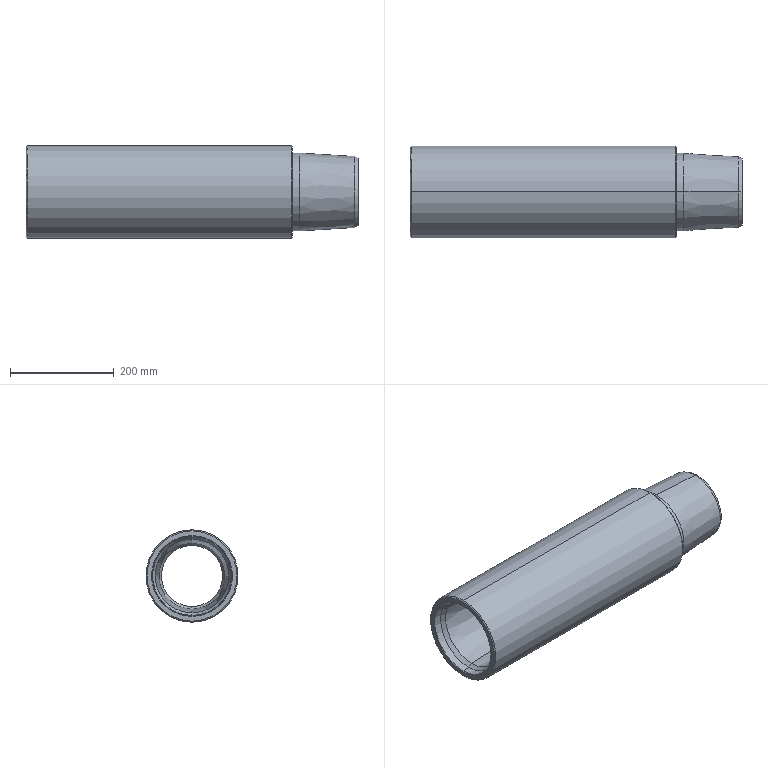Component | SolidWorks | 216OuterTube-1_SpringClipChamber-1 | 1 solid | 34 faces | box 640 x 178 x 178 mm | volume 7081697 mm3 | cone 20 | cylinder 10 | plane 4 | commonest cylinder face diameters 118 x4 150 x2 128 x2 178 x2 | material Alloy Steel
build123d program:
from build123d import *


with BuildPart() as part:
    # Model → Revolve1 (revolve)
    with BuildSketch(Plane.XY, mode=Mode.PRIVATE) as revolve1_sk:
        Polygon((512.079, 89), (3.079, 89), (1.079, 87), (1.079, 77.957), (2.077, 76.896), (17.079, 75.978), (25.583, 71.068), (143.001, 63.886), (151.465, 59), (341.079, 59), (341.079, 64), (421.079, 64), (439.739, 59), (641.079, 59), (641.079, 65.053), (635.079, 68.517), (529.079, 75), (514.079, 75), (514.079, 87), align=None)
    revolve(revolve1_sk.sketch.rotate(Axis((0, 0, 0), (1, 0, 0)), 90), axis=Axis((0, 0, 0), (1, 0, 0)))


solid = part.part
STEP:
#1=COLOUR_RGB('',0.7922,0.8196,0.9333);
#2=FILL_AREA_STYLE_COLOUR('',#1);
#3=FILL_AREA_STYLE('',(#2));
#4=SURFACE_STYLE_FILL_AREA(#3);
#5=SURFACE_SIDE_STYLE('',(#4));
#6=SURFACE_STYLE_USAGE(.BOTH.,#5);
#7=PRESENTATION_STYLE_ASSIGNMENT((#6));
#8=CARTESIAN_POINT('',(20.83,-0.,2.953));
#9=VERTEX_POINT('',#8);
#10=CARTESIAN_POINT('',(20.83,0.,-2.953));
#11=VERTEX_POINT('',#10);
#12=CARTESIAN_POINT('',(20.83,-0.,0.));
#13=DIRECTION('',(-1.,0.,0.));
#14=DIRECTION('',(0.,0.,1.));
#15=AXIS2_PLACEMENT_3D('',#12,#13,#14);
#16=CIRCLE('',#15,2.953);
#17=EDGE_CURVE('',#9,#11,#16,.T.);
#18=ORIENTED_EDGE('',*,*,#17,.T.);
#19=CARTESIAN_POINT('',(20.239,0.,-2.953));
#20=VERTEX_POINT('',#19);
#21=CARTESIAN_POINT('',(-0.,0.,-2.953));
#22=DIRECTION('',(-1.,0.,0.));
#23=VECTOR('',#22,39.37);
#24=LINE('',#21,#23);
#25=EDGE_CURVE('',#11,#20,#24,.T.);
#26=ORIENTED_EDGE('',*,*,#25,.T.);
#27=CARTESIAN_POINT('',(20.239,-0.,2.953));
#28=VERTEX_POINT('',#27);
#29=CARTESIAN_POINT('',(20.239,-0.,0.));
#30=DIRECTION('',(-1.,0.,0.));
#31=DIRECTION('',(0.,0.,1.));
#32=AXIS2_PLACEMENT_3D('',#29,#30,#31);
#33=CIRCLE('',#32,2.953);
#34=EDGE_CURVE('',#28,#20,#33,.T.);
#35=ORIENTED_EDGE('',*,*,#34,.F.);
#36=CARTESIAN_POINT('',(-0.,-0.,2.953));
#37=DIRECTION('',(-1.,0.,0.));
#38=VECTOR('',#37,39.37);
#39=LINE('',#36,#38);
#40=EDGE_CURVE('',#9,#28,#39,.T.);
#41=ORIENTED_EDGE('',*,*,#40,.F.);
#42=EDGE_LOOP('',(#18,#26,#35,#41));
#43=FACE_OUTER_BOUND('',#42,.T.);
#44=CARTESIAN_POINT('',(-0.,-0.,0.));
#45=DIRECTION('',(-1.,0.,0.));
#46=DIRECTION('',(0.,0.,1.));
#47=AXIS2_PLACEMENT_3D('',#44,#45,#46);
#48=CYLINDRICAL_SURFACE('',#47,2.953);
#49=ADVANCED_FACE('',(#43),#48,.T.);
#50=CARTESIAN_POINT('',(25.003,-0.,2.698));
#51=VERTEX_POINT('',#50);
#52=CARTESIAN_POINT('',(25.003,0.,-2.698));
#53=VERTEX_POINT('',#52);
#54=CARTESIAN_POINT('',(25.003,-0.,0.));
#55=DIRECTION('',(-1.,0.,0.));
#56=DIRECTION('',(0.,0.,1.));
#57=AXIS2_PLACEMENT_3D('',#54,#55,#56);
#58=CIRCLE('',#57,2.698);
#59=EDGE_CURVE('',#51,#53,#58,.T.);
#60=ORIENTED_EDGE('',*,*,#59,.T.);
#61=CARTESIAN_POINT('',(25.003,0.,-2.698));
#62=DIRECTION('',(-0.9981,0.,-0.06105));
#63=VECTOR('',#62,39.37);
#64=LINE('',#61,#63);
#65=EDGE_CURVE('',#53,#11,#64,.T.);
#66=ORIENTED_EDGE('',*,*,#65,.T.);
#67=ORIENTED_EDGE('',*,*,#17,.F.);
#68=CARTESIAN_POINT('',(25.003,-0.,2.698));
#69=DIRECTION('',(-0.9981,0.,0.06105));
#70=VECTOR('',#69,39.37);
#71=LINE('',#68,#70);
#72=EDGE_CURVE('',#51,#9,#71,.T.);
#73=ORIENTED_EDGE('',*,*,#72,.F.);
#74=EDGE_LOOP('',(#60,#66,#67,#73));
#75=FACE_OUTER_BOUND('',#74,.T.);
#76=CARTESIAN_POINT('',(25.003,-0.,0.));
#77=DIRECTION('',(-1.,0.,0.));
#78=DIRECTION('',(0.,0.,1.));
#79=AXIS2_PLACEMENT_3D('',#76,#77,#78);
#80=CONICAL_SURFACE('',#79,2.698,0.06109);
#81=ADVANCED_FACE('',(#75),#80,.T.);
#82=CARTESIAN_POINT('',(25.239,-0.,2.561));
#83=VERTEX_POINT('',#82);
#84=CARTESIAN_POINT('',(25.239,0.,-2.561));
#85=VERTEX_POINT('',#84);
#86=CARTESIAN_POINT('',(25.239,-0.,0.));
#87=DIRECTION('',(-1.,0.,0.));
#88=DIRECTION('',(0.,0.,1.));
#89=AXIS2_PLACEMENT_3D('',#86,#87,#88);
#90=CIRCLE('',#89,2.561);
#91=EDGE_CURVE('',#83,#85,#90,.T.);
#92=ORIENTED_EDGE('',*,*,#91,.T.);
#93=CARTESIAN_POINT('',(25.003,0.,-2.698));
#94=DIRECTION('',(-0.866,0.,-0.5));
#95=VECTOR('',#94,39.37);
#96=LINE('',#93,#95);
#97=EDGE_CURVE('',#85,#53,#96,.T.);
#98=ORIENTED_EDGE('',*,*,#97,.T.);
#99=ORIENTED_EDGE('',*,*,#59,.F.);
#100=CARTESIAN_POINT('',(25.003,-0.,2.698));
#101=DIRECTION('',(-0.866,0.,0.5));
#102=VECTOR('',#101,39.37);
#103=LINE('',#100,#102);
#104=EDGE_CURVE('',#83,#51,#103,.T.);
#105=ORIENTED_EDGE('',*,*,#104,.F.);
#106=EDGE_LOOP('',(#92,#98,#99,#105));
#107=FACE_OUTER_BOUND('',#106,.T.);
#108=CARTESIAN_POINT('',(25.003,-0.,0.));
#109=DIRECTION('',(-1.,0.,0.));
#110=DIRECTION('',(0.,0.,1.));
#111=AXIS2_PLACEMENT_3D('',#108,#109,#110);
#112=CONICAL_SURFACE('',#111,2.698,0.5236);
#113=ADVANCED_FACE('',(#107),#112,.T.);
#114=CARTESIAN_POINT('',(25.239,0.,-2.323));
#115=VERTEX_POINT('',#114);
#116=CARTESIAN_POINT('',(25.239,-0.,2.323));
#117=VERTEX_POINT('',#116);
#118=CARTESIAN_POINT('',(25.239,-0.,0.));
#119=DIRECTION('',(-1.,0.,0.));
#120=DIRECTION('',(0.,0.,1.));
#121=AXIS2_PLACEMENT_3D('',#118,#119,#120);
#122=CIRCLE('',#121,2.323);
#123=EDGE_CURVE('',#115,#117,#122,.T.);
#124=ORIENTED_EDGE('',*,*,#123,.F.);
#125=CARTESIAN_POINT('',(17.313,0.,-2.323));
#126=VERTEX_POINT('',#125);
#127=CARTESIAN_POINT('',(-0.,0.,-2.323));
#128=DIRECTION('',(-1.,0.,0.));
#129=VECTOR('',#128,39.37);
#130=LINE('',#127,#129);
#131=EDGE_CURVE('',#115,#126,#130,.T.);
#132=ORIENTED_EDGE('',*,*,#131,.T.);
#133=CARTESIAN_POINT('',(17.313,-0.,2.323));
#134=VERTEX_POINT('',#133);
#135=CARTESIAN_POINT('',(17.313,-0.,0.));
#136=DIRECTION('',(-1.,0.,0.));
#137=DIRECTION('',(0.,0.,1.));
#138=AXIS2_PLACEMENT_3D('',#135,#136,#137);
#139=CIRCLE('',#138,2.323);
#140=EDGE_CURVE('',#126,#134,#139,.T.);
#141=ORIENTED_EDGE('',*,*,#140,.T.);
#142=CARTESIAN_POINT('',(-0.,-0.,2.323));
#143=DIRECTION('',(-1.,0.,0.));
#144=VECTOR('',#143,39.37);
#145=LINE('',#142,#144);
#146=EDGE_CURVE('',#117,#134,#145,.T.);
#147=ORIENTED_EDGE('',*,*,#146,.F.);
#148=EDGE_LOOP('',(#124,#132,#141,#147));
#149=FACE_OUTER_BOUND('',#148,.T.);
#150=CARTESIAN_POINT('',(-0.,-0.,0.));
#151=DIRECTION('',(-1.,0.,0.));
#152=DIRECTION('',(0.,0.,1.));
#153=AXIS2_PLACEMENT_3D('',#150,#151,#152);
#154=CYLINDRICAL_SURFACE('',#153,2.323);
#155=ADVANCED_FACE('',(#149),#154,.F.);
#156=ORIENTED_EDGE('',*,*,#140,.F.);
#157=CARTESIAN_POINT('',(16.578,0.,-2.52));
#158=VERTEX_POINT('',#157);
#159=CARTESIAN_POINT('',(16.578,0.,-2.52));
#160=DIRECTION('',(-0.9659,0.,-0.2588));
#161=VECTOR('',#160,39.37);
#162=LINE('',#159,#161);
#163=EDGE_CURVE('',#126,#158,#162,.T.);
#164=ORIENTED_EDGE('',*,*,#163,.T.);
#165=CARTESIAN_POINT('',(16.578,-0.,2.52));
#166=VERTEX_POINT('',#165);
#167=CARTESIAN_POINT('',(16.578,-0.,0.));
#168=DIRECTION('',(-1.,0.,0.));
#169=DIRECTION('',(0.,0.,1.));
#170=AXIS2_PLACEMENT_3D('',#167,#168,#169);
#171=CIRCLE('',#170,2.52);
#172=EDGE_CURVE('',#158,#166,#171,.T.);
#173=ORIENTED_EDGE('',*,*,#172,.T.);
#174=CARTESIAN_POINT('',(16.578,-0.,2.52));
#175=DIRECTION('',(-0.9659,0.,0.2588));
#176=VECTOR('',#175,39.37);
#177=LINE('',#174,#176);
#178=EDGE_CURVE('',#134,#166,#177,.T.);
#179=ORIENTED_EDGE('',*,*,#178,.F.);
#180=EDGE_LOOP('',(#156,#164,#173,#179));
#181=FACE_OUTER_BOUND('',#180,.T.);
#182=CARTESIAN_POINT('',(16.578,-0.,0.));
#183=DIRECTION('',(-1.,0.,0.));
#184=DIRECTION('',(0.,0.,1.));
#185=AXIS2_PLACEMENT_3D('',#182,#183,#184);
#186=CONICAL_SURFACE('',#185,2.52,0.2618);
#187=ADVANCED_FACE('',(#181),#186,.F.);
#188=ORIENTED_EDGE('',*,*,#172,.F.);
#189=CARTESIAN_POINT('',(13.428,0.,-2.52));
#190=VERTEX_POINT('',#189);
#191=CARTESIAN_POINT('',(-0.,0.,-2.52));
#192=DIRECTION('',(-1.,0.,0.));
#193=VECTOR('',#192,39.37);
#194=LINE('',#191,#193);
#195=EDGE_CURVE('',#158,#190,#194,.T.);
#196=ORIENTED_EDGE('',*,*,#195,.T.);
#197=CARTESIAN_POINT('',(13.428,-0.,2.52));
#198=VERTEX_POINT('',#197);
#199=CARTESIAN_POINT('',(13.428,-0.,0.));
#200=DIRECTION('',(-1.,0.,0.));
#201=DIRECTION('',(0.,0.,1.));
#202=AXIS2_PLACEMENT_3D('',#199,#200,#201);
#203=CIRCLE('',#202,2.52);
#204=EDGE_CURVE('',#190,#198,#203,.T.);
#205=ORIENTED_EDGE('',*,*,#204,.T.);
#206=CARTESIAN_POINT('',(-0.,-0.,2.52));
#207=DIRECTION('',(-1.,0.,0.));
#208=VECTOR('',#207,39.37);
#209=LINE('',#206,#208);
#210=EDGE_CURVE('',#166,#198,#209,.T.);
#211=ORIENTED_EDGE('',*,*,#210,.F.);
#212=EDGE_LOOP('',(#188,#196,#205,#211));
#213=FACE_OUTER_BOUND('',#212,.T.);
#214=CARTESIAN_POINT('',(-0.,-0.,0.));
#215=DIRECTION('',(-1.,0.,0.));
#216=DIRECTION('',(0.,0.,1.));
#217=AXIS2_PLACEMENT_3D('',#214,#215,#216);
#218=CYLINDRICAL_SURFACE('',#217,2.52);
#219=ADVANCED_FACE('',(#213),#218,.F.);
#220=CARTESIAN_POINT('',(13.428,0.,-2.323));
#221=VERTEX_POINT('',#220);
#222=CARTESIAN_POINT('',(13.428,-0.,2.323));
#223=VERTEX_POINT('',#222);
#224=CARTESIAN_POINT('',(13.428,-0.,0.));
#225=DIRECTION('',(-1.,0.,0.));
#226=DIRECTION('',(0.,0.,1.));
#227=AXIS2_PLACEMENT_3D('',#224,#225,#226);
#228=CIRCLE('',#227,2.323);
#229=EDGE_CURVE('',#221,#223,#228,.T.);
#230=ORIENTED_EDGE('',*,*,#229,.F.);
#231=CARTESIAN_POINT('',(5.963,0.,-2.323));
#232=VERTEX_POINT('',#231);
#233=CARTESIAN_POINT('',(-0.,0.,-2.323));
#234=DIRECTION('',(-1.,0.,0.));
#235=VECTOR('',#234,39.37);
#236=LINE('',#233,#235);
#237=EDGE_CURVE('',#221,#232,#236,.T.);
#238=ORIENTED_EDGE('',*,*,#237,.T.);
#239=CARTESIAN_POINT('',(5.963,-0.,2.323));
#240=VERTEX_POINT('',#239);
#241=CARTESIAN_POINT('',(5.963,-0.,0.));
#242=DIRECTION('',(-1.,0.,0.));
#243=DIRECTION('',(0.,0.,1.));
#244=AXIS2_PLACEMENT_3D('',#241,#242,#243);
#245=CIRCLE('',#244,2.323);
#246=EDGE_CURVE('',#232,#240,#245,.T.);
#247=ORIENTED_EDGE('',*,*,#246,.T.);
#248=CARTESIAN_POINT('',(-0.,-0.,2.323));
#249=DIRECTION('',(-1.,0.,0.));
#250=VECTOR('',#249,39.37);
#251=LINE('',#248,#250);
#252=EDGE_CURVE('',#223,#240,#251,.T.);
#253=ORIENTED_EDGE('',*,*,#252,.F.);
#254=EDGE_LOOP('',(#230,#238,#247,#253));
#255=FACE_OUTER_BOUND('',#254,.T.);
#256=CARTESIAN_POINT('',(-0.,-0.,0.));
#257=DIRECTION('',(-1.,0.,0.));
#258=DIRECTION('',(0.,0.,1.));
#259=AXIS2_PLACEMENT_3D('',#256,#257,#258);
#260=CYLINDRICAL_SURFACE('',#259,2.323);
#261=ADVANCED_FACE('',(#255),#260,.F.);
#262=ORIENTED_EDGE('',*,*,#246,.F.);
#263=CARTESIAN_POINT('',(5.63,0.,-2.515));
#264=VERTEX_POINT('',#263);
#265=CARTESIAN_POINT('',(5.63,0.,-2.515));
#266=DIRECTION('',(-0.866,0.,-0.5));
#267=VECTOR('',#266,39.37);
#268=LINE('',#265,#267);
#269=EDGE_CURVE('',#232,#264,#268,.T.);
#270=ORIENTED_EDGE('',*,*,#269,.T.);
#271=CARTESIAN_POINT('',(5.63,-0.,2.515));
#272=VERTEX_POINT('',#271);
#273=CARTESIAN_POINT('',(5.63,-0.,0.));
#274=DIRECTION('',(-1.,0.,0.));
#275=DIRECTION('',(0.,0.,1.));
#276=AXIS2_PLACEMENT_3D('',#273,#274,#275);
#277=CIRCLE('',#276,2.515);
#278=EDGE_CURVE('',#264,#272,#277,.T.);
#279=ORIENTED_EDGE('',*,*,#278,.T.);
#280=CARTESIAN_POINT('',(5.63,-0.,2.515));
#281=DIRECTION('',(-0.866,0.,0.5));
#282=VECTOR('',#281,39.37);
#283=LINE('',#280,#282);
#284=EDGE_CURVE('',#240,#272,#283,.T.);
#285=ORIENTED_EDGE('',*,*,#284,.F.);
#286=EDGE_LOOP('',(#262,#270,#279,#285));
#287=FACE_OUTER_BOUND('',#286,.T.);
#288=CARTESIAN_POINT('',(5.63,-0.,0.));
#289=DIRECTION('',(-1.,0.,0.));
#290=DIRECTION('',(0.,0.,1.));
#291=AXIS2_PLACEMENT_3D('',#288,#289,#290);
#292=CONICAL_SURFACE('',#291,2.515,0.5236);
#293=ADVANCED_FACE('',(#287),#292,.F.);
#294=ORIENTED_EDGE('',*,*,#278,.F.);
#295=CARTESIAN_POINT('',(1.007,0.,-2.798));
#296=VERTEX_POINT('',#295);
#297=CARTESIAN_POINT('',(1.007,0.,-2.798));
#298=DIRECTION('',(-0.9981,0.,-0.06105));
#299=VECTOR('',#298,39.37);
#300=LINE('',#297,#299);
#301=EDGE_CURVE('',#264,#296,#300,.T.);
#302=ORIENTED_EDGE('',*,*,#301,.T.);
#303=CARTESIAN_POINT('',(1.007,-0.,2.798));
#304=VERTEX_POINT('',#303);
#305=CARTESIAN_POINT('',(1.007,-0.,0.));
#306=DIRECTION('',(-1.,0.,0.));
#307=DIRECTION('',(0.,0.,1.));
#308=AXIS2_PLACEMENT_3D('',#305,#306,#307);
#309=CIRCLE('',#308,2.798);
#310=EDGE_CURVE('',#296,#304,#309,.T.);
#311=ORIENTED_EDGE('',*,*,#310,.T.);
#312=CARTESIAN_POINT('',(1.007,-0.,2.798));
#313=DIRECTION('',(-0.9981,0.,0.06105));
#314=VECTOR('',#313,39.37);
#315=LINE('',#312,#314);
#316=EDGE_CURVE('',#272,#304,#315,.T.);
#317=ORIENTED_EDGE('',*,*,#316,.F.);
#318=EDGE_LOOP('',(#294,#302,#311,#317));
#319=FACE_OUTER_BOUND('',#318,.T.);
#320=CARTESIAN_POINT('',(1.007,-0.,0.));
#321=DIRECTION('',(-1.,0.,0.));
#322=DIRECTION('',(0.,0.,1.));
#323=AXIS2_PLACEMENT_3D('',#320,#321,#322);
#324=CONICAL_SURFACE('',#323,2.798,0.06109);
#325=ADVANCED_FACE('',(#319),#324,.F.);
#326=ORIENTED_EDGE('',*,*,#310,.F.);
#327=CARTESIAN_POINT('',(0.6724,0.,-2.991));
#328=VERTEX_POINT('',#327);
#329=CARTESIAN_POINT('',(0.6724,0.,-2.991));
#330=DIRECTION('',(-0.866,0.,-0.5));
#331=VECTOR('',#330,39.37);
#332=LINE('',#329,#331);
#333=EDGE_CURVE('',#296,#328,#332,.T.);
#334=ORIENTED_EDGE('',*,*,#333,.T.);
#335=CARTESIAN_POINT('',(0.6724,-0.,2.991));
#336=VERTEX_POINT('',#335);
#337=CARTESIAN_POINT('',(0.6724,-0.,0.));
#338=DIRECTION('',(-1.,0.,0.));
#339=DIRECTION('',(0.,0.,1.));
#340=AXIS2_PLACEMENT_3D('',#337,#338,#339);
#341=CIRCLE('',#340,2.991);
#342=EDGE_CURVE('',#328,#336,#341,.T.);
#343=ORIENTED_EDGE('',*,*,#342,.T.);
#344=CARTESIAN_POINT('',(0.6724,-0.,2.991));
#345=DIRECTION('',(-0.866,0.,0.5));
#346=VECTOR('',#345,39.37);
#347=LINE('',#344,#346);
#348=EDGE_CURVE('',#304,#336,#347,.T.);
#349=ORIENTED_EDGE('',*,*,#348,.F.);
#350=EDGE_LOOP('',(#326,#334,#343,#349));
#351=FACE_OUTER_BOUND('',#350,.T.);
#352=CARTESIAN_POINT('',(0.6724,-0.,0.));
#353=DIRECTION('',(-1.,0.,0.));
#354=DIRECTION('',(0.,0.,1.));
#355=AXIS2_PLACEMENT_3D('',#352,#353,#354);
#356=CONICAL_SURFACE('',#355,2.991,0.5236);
#357=ADVANCED_FACE('',(#351),#356,.F.);
#358=ORIENTED_EDGE('',*,*,#342,.F.);
#359=CARTESIAN_POINT('',(0.08177,0.,-3.027));
#360=VERTEX_POINT('',#359);
#361=CARTESIAN_POINT('',(0.08177,0.,-3.027));
#362=DIRECTION('',(-0.9981,0.,-0.06105));
#363=VECTOR('',#362,39.37);
#364=LINE('',#361,#363);
#365=EDGE_CURVE('',#328,#360,#364,.T.);
#366=ORIENTED_EDGE('',*,*,#365,.T.);
#367=CARTESIAN_POINT('',(0.08177,-0.,3.027));
#368=VERTEX_POINT('',#367);
#369=CARTESIAN_POINT('',(0.08177,-0.,0.));
#370=DIRECTION('',(-1.,0.,0.));
#371=DIRECTION('',(0.,0.,1.));
#372=AXIS2_PLACEMENT_3D('',#369,#370,#371);
#373=CIRCLE('',#372,3.027);
#374=EDGE_CURVE('',#360,#368,#373,.T.);
#375=ORIENTED_EDGE('',*,*,#374,.T.);
#376=CARTESIAN_POINT('',(0.08177,-0.,3.027));
#377=DIRECTION('',(-0.9981,0.,0.06105));
#378=VECTOR('',#377,39.37);
#379=LINE('',#376,#378);
#380=EDGE_CURVE('',#336,#368,#379,.T.);
#381=ORIENTED_EDGE('',*,*,#380,.F.);
#382=EDGE_LOOP('',(#358,#366,#375,#381));
#383=FACE_OUTER_BOUND('',#382,.T.);
#384=CARTESIAN_POINT('',(0.08177,-0.,0.));
#385=DIRECTION('',(-1.,0.,0.));
#386=DIRECTION('',(0.,0.,1.));
#387=AXIS2_PLACEMENT_3D('',#384,#385,#386);
#388=CONICAL_SURFACE('',#387,3.027,0.06109);
#389=ADVANCED_FACE('',(#383),#388,.F.);
#390=ORIENTED_EDGE('',*,*,#374,.F.);
#391=CARTESIAN_POINT('',(0.04247,0.,-3.069));
#392=VERTEX_POINT('',#391);
#393=CARTESIAN_POINT('',(0.04247,0.,-3.069));
#394=DIRECTION('',(-0.6852,0.,-0.7284));
#395=VECTOR('',#394,39.37);
#396=LINE('',#393,#395);
#397=EDGE_CURVE('',#360,#392,#396,.T.);
#398=ORIENTED_EDGE('',*,*,#397,.T.);
#399=CARTESIAN_POINT('',(0.04247,-0.,3.069));
#400=VERTEX_POINT('',#399);
#401=CARTESIAN_POINT('',(0.04247,-0.,0.));
#402=DIRECTION('',(-1.,0.,0.));
#403=DIRECTION('',(0.,0.,1.));
#404=AXIS2_PLACEMENT_3D('',#401,#402,#403);
#405=CIRCLE('',#404,3.069);
#406=EDGE_CURVE('',#392,#400,#405,.T.);
#407=ORIENTED_EDGE('',*,*,#406,.T.);
#408=CARTESIAN_POINT('',(0.04247,-0.,3.069));
#409=DIRECTION('',(-0.6852,0.,0.7284));
#410=VECTOR('',#409,39.37);
#411=LINE('',#408,#410);
#412=EDGE_CURVE('',#368,#400,#411,.T.);
#413=ORIENTED_EDGE('',*,*,#412,.F.);
#414=EDGE_LOOP('',(#390,#398,#407,#413));
#415=FACE_OUTER_BOUND('',#414,.T.);
#416=CARTESIAN_POINT('',(0.04247,-0.,0.));
#417=DIRECTION('',(-1.,0.,0.));
#418=DIRECTION('',(0.,0.,1.));
#419=AXIS2_PLACEMENT_3D('',#416,#417,#418);
#420=CONICAL_SURFACE('',#419,3.069,0.8159);
#421=ADVANCED_FACE('',(#415),#420,.F.);
#422=CARTESIAN_POINT('',(0.04247,0.,3.425));
#423=VERTEX_POINT('',#422);
#424=CARTESIAN_POINT('',(0.04247,-0.,-3.425));
#425=VERTEX_POINT('',#424);
#426=CARTESIAN_POINT('',(0.04247,-0.,0.));
#427=DIRECTION('',(-1.,0.,0.));
#428=DIRECTION('',(0.,0.,1.));
#429=AXIS2_PLACEMENT_3D('',#426,#427,#428);
#430=CIRCLE('',#429,3.425);
#431=EDGE_CURVE('',#423,#425,#430,.T.);
#432=ORIENTED_EDGE('',*,*,#431,.F.);
#433=CARTESIAN_POINT('',(0.1212,-0.,3.504));
#434=VERTEX_POINT('',#433);
#435=CARTESIAN_POINT('',(0.04247,0.,3.425));
#436=DIRECTION('',(0.7071,0.,0.7071));
#437=VECTOR('',#436,39.37);
#438=LINE('',#435,#437);
#439=EDGE_CURVE('',#423,#434,#438,.T.);
#440=ORIENTED_EDGE('',*,*,#439,.T.);
#441=CARTESIAN_POINT('',(0.1212,0.,-3.504));
#442=VERTEX_POINT('',#441);
#443=CARTESIAN_POINT('',(0.1212,-0.,0.));
#444=DIRECTION('',(-1.,0.,0.));
#445=DIRECTION('',(0.,0.,1.));
#446=AXIS2_PLACEMENT_3D('',#443,#444,#445);
#447=CIRCLE('',#446,3.504);
#448=EDGE_CURVE('',#434,#442,#447,.T.);
#449=ORIENTED_EDGE('',*,*,#448,.T.);
#450=CARTESIAN_POINT('',(0.04247,-0.,-3.425));
#451=DIRECTION('',(0.7071,0.,-0.7071));
#452=VECTOR('',#451,39.37);
#453=LINE('',#450,#452);
#454=EDGE_CURVE('',#425,#442,#453,.T.);
#455=ORIENTED_EDGE('',*,*,#454,.F.);
#456=EDGE_LOOP('',(#432,#440,#449,#455));
#457=FACE_OUTER_BOUND('',#456,.T.);
#458=CARTESIAN_POINT('',(0.04247,-0.,0.));
#459=DIRECTION('',(1.,0.,0.));
#460=DIRECTION('',(0.,0.,-1.));
#461=AXIS2_PLACEMENT_3D('',#458,#459,#460);
#462=CONICAL_SURFACE('',#461,3.425,0.7854);
#463=ADVANCED_FACE('',(#457),#462,.T.);
#464=CARTESIAN_POINT('',(20.161,-0.,3.504));
#465=VERTEX_POINT('',#464);
#466=CARTESIAN_POINT('',(20.161,0.,-3.504));
#467=VERTEX_POINT('',#466);
#468=CARTESIAN_POINT('',(20.161,-0.,0.));
#469=DIRECTION('',(-1.,0.,0.));
#470=DIRECTION('',(0.,0.,1.));
#471=AXIS2_PLACEMENT_3D('',#468,#469,#470);
#472=CIRCLE('',#471,3.504);
#473=EDGE_CURVE('',#465,#467,#472,.T.);
#474=ORIENTED_EDGE('',*,*,#473,.T.);
#475=CARTESIAN_POINT('',(-0.,0.,-3.504));
#476=DIRECTION('',(-1.,0.,0.));
#477=VECTOR('',#476,39.37);
#478=LINE('',#475,#477);
#479=EDGE_CURVE('',#467,#442,#478,.T.);
#480=ORIENTED_EDGE('',*,*,#479,.T.);
#481=ORIENTED_EDGE('',*,*,#448,.F.);
#482=CARTESIAN_POINT('',(-0.,-0.,3.504));
#483=DIRECTION('',(-1.,0.,0.));
#484=VECTOR('',#483,39.37);
#485=LINE('',#482,#484);
#486=EDGE_CURVE('',#465,#434,#485,.T.);
#487=ORIENTED_EDGE('',*,*,#486,.F.);
#488=EDGE_LOOP('',(#474,#480,#481,#487));
#489=FACE_OUTER_BOUND('',#488,.T.);
#490=CARTESIAN_POINT('',(-0.,-0.,0.));
#491=DIRECTION('',(-1.,0.,0.));
#492=DIRECTION('',(0.,0.,1.));
#493=AXIS2_PLACEMENT_3D('',#490,#491,#492);
#494=CYLINDRICAL_SURFACE('',#493,3.504);
#495=ADVANCED_FACE('',(#489),#494,.T.);
#496=CARTESIAN_POINT('',(20.239,-0.,3.425));
#497=VERTEX_POINT('',#496);
#498=CARTESIAN_POINT('',(20.239,0.,-3.425));
#499=VERTEX_POINT('',#498);
#500=CARTESIAN_POINT('',(20.239,-0.,0.));
#501=DIRECTION('',(-1.,0.,0.));
#502=DIRECTION('',(0.,0.,1.));
#503=AXIS2_PLACEMENT_3D('',#500,#501,#502);
#504=CIRCLE('',#503,3.425);
#505=EDGE_CURVE('',#497,#499,#504,.T.);
#506=ORIENTED_EDGE('',*,*,#505,.T.);
#507=CARTESIAN_POINT('',(20.239,0.,-3.425));
#508=DIRECTION('',(-0.7071,0.,-0.7071));
#509=VECTOR('',#508,39.37);
#510=LINE('',#507,#509);
#511=EDGE_CURVE('',#499,#467,#510,.T.);
#512=ORIENTED_EDGE('',*,*,#511,.T.);
#513=ORIENTED_EDGE('',*,*,#473,.F.);
#514=CARTESIAN_POINT('',(20.239,-0.,3.425));
#515=DIRECTION('',(-0.7071,0.,0.7071));
#516=VECTOR('',#515,39.37);
#517=LINE('',#514,#516);
#518=EDGE_CURVE('',#497,#465,#517,.T.);
#519=ORIENTED_EDGE('',*,*,#518,.F.);
#520=EDGE_LOOP('',(#506,#512,#513,#519));
#521=FACE_OUTER_BOUND('',#520,.T.);
#522=CARTESIAN_POINT('',(20.239,-0.,0.));
#523=DIRECTION('',(-1.,0.,0.));
#524=DIRECTION('',(0.,0.,1.));
#525=AXIS2_PLACEMENT_3D('',#522,#523,#524);
#526=CONICAL_SURFACE('',#525,3.425,0.7854);
#527=ADVANCED_FACE('',(#521),#526,.T.);
#528=ORIENTED_EDGE('',*,*,#34,.T.);
#529=CARTESIAN_POINT('',(20.239,-0.,0.));
#530=DIRECTION('',(-1.,0.,0.));
#531=DIRECTION('',(0.,0.,1.));
#532=AXIS2_PLACEMENT_3D('',#529,#530,#531);
#533=CIRCLE('',#532,2.953);
#534=EDGE_CURVE('',#20,#28,#533,.T.);
#535=ORIENTED_EDGE('',*,*,#534,.T.);
#536=EDGE_LOOP('',(#528,#535));
#537=FACE_BOUND('',#536,.T.);
#538=ORIENTED_EDGE('',*,*,#505,.F.);
#539=CARTESIAN_POINT('',(20.239,-0.,0.));
#540=DIRECTION('',(-1.,0.,0.));
#541=DIRECTION('',(0.,0.,1.));
#542=AXIS2_PLACEMENT_3D('',#539,#540,#541);
#543=CIRCLE('',#542,3.425);
#544=EDGE_CURVE('',#499,#497,#543,.T.);
#545=ORIENTED_EDGE('',*,*,#544,.F.);
#546=EDGE_LOOP('',(#538,#545));
#547=FACE_OUTER_BOUND('',#546,.T.);
#548=CARTESIAN_POINT('',(20.239,0.,0.));
#549=DIRECTION('',(1.,0.,0.));
#550=DIRECTION('',(0.,0.,-1.));
#551=AXIS2_PLACEMENT_3D('',#548,#549,#550);
#552=PLANE('',#551);
#553=ADVANCED_FACE('',(#537,#547),#552,.T.);
#554=ORIENTED_EDGE('',*,*,#511,.F.);
#555=ORIENTED_EDGE('',*,*,#544,.T.);
#556=ORIENTED_EDGE('',*,*,#518,.T.);
#557=CARTESIAN_POINT('',(20.161,-0.,0.));
#558=DIRECTION('',(-1.,0.,0.));
#559=DIRECTION('',(0.,0.,1.));
#560=AXIS2_PLACEMENT_3D('',#557,#558,#559);
#561=CIRCLE('',#560,3.504);
#562=EDGE_CURVE('',#467,#465,#561,.T.);
#563=ORIENTED_EDGE('',*,*,#562,.F.);
#564=EDGE_LOOP('',(#554,#555,#556,#563));
#565=FACE_OUTER_BOUND('',#564,.T.);
#566=CARTESIAN_POINT('',(20.239,-0.,0.));
#567=DIRECTION('',(-1.,0.,0.));
#568=DIRECTION('',(0.,0.,1.));
#569=AXIS2_PLACEMENT_3D('',#566,#567,#568);
#570=CONICAL_SURFACE('',#569,3.425,0.7854);
#571=ADVANCED_FACE('',(#565),#570,.T.);
#572=ORIENTED_EDGE('',*,*,#479,.F.);
#573=ORIENTED_EDGE('',*,*,#562,.T.);
#574=ORIENTED_EDGE('',*,*,#486,.T.);
#575=CARTESIAN_POINT('',(0.1212,-0.,0.));
#576=DIRECTION('',(-1.,0.,0.));
#577=DIRECTION('',(0.,0.,1.));
#578=AXIS2_PLACEMENT_3D('',#575,#576,#577);
#579=CIRCLE('',#578,3.504);
#580=EDGE_CURVE('',#442,#434,#579,.T.);
#581=ORIENTED_EDGE('',*,*,#580,.F.);
#582=EDGE_LOOP('',(#572,#573,#574,#581));
#583=FACE_OUTER_BOUND('',#582,.T.);
#584=CARTESIAN_POINT('',(-0.,-0.,0.));
#585=DIRECTION('',(-1.,0.,0.));
#586=DIRECTION('',(0.,0.,1.));
#587=AXIS2_PLACEMENT_3D('',#584,#585,#586);
#588=CYLINDRICAL_SURFACE('',#587,3.504);
#589=ADVANCED_FACE('',(#583),#588,.T.);
#590=ORIENTED_EDGE('',*,*,#439,.F.);
#591=CARTESIAN_POINT('',(0.04247,-0.,0.));
#592=DIRECTION('',(-1.,0.,0.));
#593=DIRECTION('',(0.,0.,1.));
#594=AXIS2_PLACEMENT_3D('',#591,#592,#593);
#595=CIRCLE('',#594,3.425);
#596=EDGE_CURVE('',#425,#423,#595,.T.);
#597=ORIENTED_EDGE('',*,*,#596,.F.);
#598=ORIENTED_EDGE('',*,*,#454,.T.);
#599=ORIENTED_EDGE('',*,*,#580,.T.);
#600=EDGE_LOOP('',(#590,#597,#598,#599));
#601=FACE_OUTER_BOUND('',#600,.T.);
#602=CARTESIAN_POINT('',(0.04247,-0.,0.));
#603=DIRECTION('',(1.,0.,0.));
#604=DIRECTION('',(0.,0.,-1.));
#605=AXIS2_PLACEMENT_3D('',#602,#603,#604);
#606=CONICAL_SURFACE('',#605,3.425,0.7854);
#607=ADVANCED_FACE('',(#601),#606,.T.);
#608=ORIENTED_EDGE('',*,*,#596,.T.);
#609=ORIENTED_EDGE('',*,*,#431,.T.);
#610=EDGE_LOOP('',(#608,#609));
#611=FACE_OUTER_BOUND('',#610,.T.);
#612=CARTESIAN_POINT('',(0.04247,-0.,0.));
#613=DIRECTION('',(-1.,0.,0.));
#614=DIRECTION('',(0.,0.,1.));
#615=AXIS2_PLACEMENT_3D('',#612,#613,#614);
#616=CIRCLE('',#615,3.069);
#617=EDGE_CURVE('',#400,#392,#616,.T.);
#618=ORIENTED_EDGE('',*,*,#617,.F.);
#619=ORIENTED_EDGE('',*,*,#406,.F.);
#620=EDGE_LOOP('',(#618,#619));
#621=FACE_BOUND('',#620,.T.);
#622=CARTESIAN_POINT('',(0.04247,0.,0.));
#623=DIRECTION('',(-1.,0.,0.));
#624=DIRECTION('',(0.,0.,1.));
#625=AXIS2_PLACEMENT_3D('',#622,#623,#624);
#626=PLANE('',#625);
#627=ADVANCED_FACE('',(#611,#621),#626,.T.);
#628=ORIENTED_EDGE('',*,*,#397,.F.);
#629=CARTESIAN_POINT('',(0.08177,-0.,0.));
#630=DIRECTION('',(-1.,0.,0.));
#631=DIRECTION('',(0.,0.,1.));
#632=AXIS2_PLACEMENT_3D('',#629,#630,#631);
#633=CIRCLE('',#632,3.027);
#634=EDGE_CURVE('',#368,#360,#633,.T.);
#635=ORIENTED_EDGE('',*,*,#634,.F.);
#636=ORIENTED_EDGE('',*,*,#412,.T.);
#637=ORIENTED_EDGE('',*,*,#617,.T.);
#638=EDGE_LOOP('',(#628,#635,#636,#637));
#639=FACE_OUTER_BOUND('',#638,.T.);
#640=CARTESIAN_POINT('',(0.04247,-0.,0.));
#641=DIRECTION('',(-1.,0.,0.));
#642=DIRECTION('',(0.,0.,1.));
#643=AXIS2_PLACEMENT_3D('',#640,#641,#642);
#644=CONICAL_SURFACE('',#643,3.069,0.8159);
#645=ADVANCED_FACE('',(#639),#644,.F.);
#646=ORIENTED_EDGE('',*,*,#365,.F.);
#647=CARTESIAN_POINT('',(0.6724,-0.,0.));
#648=DIRECTION('',(-1.,0.,0.));
#649=DIRECTION('',(0.,0.,1.));
#650=AXIS2_PLACEMENT_3D('',#647,#648,#649);
#651=CIRCLE('',#650,2.991);
#652=EDGE_CURVE('',#336,#328,#651,.T.);
#653=ORIENTED_EDGE('',*,*,#652,.F.);
#654=ORIENTED_EDGE('',*,*,#380,.T.);
#655=ORIENTED_EDGE('',*,*,#634,.T.);
#656=EDGE_LOOP('',(#646,#653,#654,#655));
#657=FACE_OUTER_BOUND('',#656,.T.);
#658=CARTESIAN_POINT('',(0.08177,-0.,0.));
#659=DIRECTION('',(-1.,0.,0.));
#660=DIRECTION('',(0.,0.,1.));
#661=AXIS2_PLACEMENT_3D('',#658,#659,#660);
#662=CONICAL_SURFACE('',#661,3.027,0.06109);
#663=ADVANCED_FACE('',(#657),#662,.F.);
#664=ORIENTED_EDGE('',*,*,#333,.F.);
#665=CARTESIAN_POINT('',(1.007,-0.,0.));
#666=DIRECTION('',(-1.,0.,0.));
#667=DIRECTION('',(0.,0.,1.));
#668=AXIS2_PLACEMENT_3D('',#665,#666,#667);
#669=CIRCLE('',#668,2.798);
#670=EDGE_CURVE('',#304,#296,#669,.T.);
#671=ORIENTED_EDGE('',*,*,#670,.F.);
#672=ORIENTED_EDGE('',*,*,#348,.T.);
#673=ORIENTED_EDGE('',*,*,#652,.T.);
#674=EDGE_LOOP('',(#664,#671,#672,#673));
#675=FACE_OUTER_BOUND('',#674,.T.);
#676=CARTESIAN_POINT('',(0.6724,-0.,0.));
#677=DIRECTION('',(-1.,0.,0.));
#678=DIRECTION('',(0.,0.,1.));
#679=AXIS2_PLACEMENT_3D('',#676,#677,#678);
#680=CONICAL_SURFACE('',#679,2.991,0.5236);
#681=ADVANCED_FACE('',(#675),#680,.F.);
#682=ORIENTED_EDGE('',*,*,#301,.F.);
#683=CARTESIAN_POINT('',(5.63,-0.,0.));
#684=DIRECTION('',(-1.,0.,0.));
#685=DIRECTION('',(0.,0.,1.));
#686=AXIS2_PLACEMENT_3D('',#683,#684,#685);
#687=CIRCLE('',#686,2.515);
#688=EDGE_CURVE('',#272,#264,#687,.T.);
#689=ORIENTED_EDGE('',*,*,#688,.F.);
#690=ORIENTED_EDGE('',*,*,#316,.T.);
#691=ORIENTED_EDGE('',*,*,#670,.T.);
#692=EDGE_LOOP('',(#682,#689,#690,#691));
#693=FACE_OUTER_BOUND('',#692,.T.);
#694=CARTESIAN_POINT('',(1.007,-0.,0.));
#695=DIRECTION('',(-1.,0.,0.));
#696=DIRECTION('',(0.,0.,1.));
#697=AXIS2_PLACEMENT_3D('',#694,#695,#696);
#698=CONICAL_SURFACE('',#697,2.798,0.06109);
#699=ADVANCED_FACE('',(#693),#698,.F.);
#700=ORIENTED_EDGE('',*,*,#269,.F.);
#701=CARTESIAN_POINT('',(5.963,-0.,0.));
#702=DIRECTION('',(-1.,0.,0.));
#703=DIRECTION('',(0.,0.,1.));
#704=AXIS2_PLACEMENT_3D('',#701,#702,#703);
#705=CIRCLE('',#704,2.323);
#706=EDGE_CURVE('',#240,#232,#705,.T.);
#707=ORIENTED_EDGE('',*,*,#706,.F.);
#708=ORIENTED_EDGE('',*,*,#284,.T.);
#709=ORIENTED_EDGE('',*,*,#688,.T.);
#710=EDGE_LOOP('',(#700,#707,#708,#709));
#711=FACE_OUTER_BOUND('',#710,.T.);
#712=CARTESIAN_POINT('',(5.63,-0.,0.));
#713=DIRECTION('',(-1.,0.,0.));
#714=DIRECTION('',(0.,0.,1.));
#715=AXIS2_PLACEMENT_3D('',#712,#713,#714);
#716=CONICAL_SURFACE('',#715,2.515,0.5236);
#717=ADVANCED_FACE('',(#711),#716,.F.);
#718=ORIENTED_EDGE('',*,*,#237,.F.);
#719=CARTESIAN_POINT('',(13.428,-0.,0.));
#720=DIRECTION('',(-1.,0.,0.));
#721=DIRECTION('',(0.,0.,1.));
#722=AXIS2_PLACEMENT_3D('',#719,#720,#721);
#723=CIRCLE('',#722,2.323);
#724=EDGE_CURVE('',#223,#221,#723,.T.);
#725=ORIENTED_EDGE('',*,*,#724,.F.);
#726=ORIENTED_EDGE('',*,*,#252,.T.);
#727=ORIENTED_EDGE('',*,*,#706,.T.);
#728=EDGE_LOOP('',(#718,#725,#726,#727));
#729=FACE_OUTER_BOUND('',#728,.T.);
#730=CARTESIAN_POINT('',(-0.,-0.,0.));
#731=DIRECTION('',(-1.,0.,0.));
#732=DIRECTION('',(0.,0.,1.));
#733=AXIS2_PLACEMENT_3D('',#730,#731,#732);
#734=CYLINDRICAL_SURFACE('',#733,2.323);
#735=ADVANCED_FACE('',(#729),#734,.F.);
#736=ORIENTED_EDGE('',*,*,#724,.T.);
#737=ORIENTED_EDGE('',*,*,#229,.T.);
#738=EDGE_LOOP('',(#736,#737));
#739=FACE_BOUND('',#738,.T.);
#740=CARTESIAN_POINT('',(13.428,-0.,0.));
#741=DIRECTION('',(-1.,0.,0.));
#742=DIRECTION('',(0.,0.,1.));
#743=AXIS2_PLACEMENT_3D('',#740,#741,#742);
#744=CIRCLE('',#743,2.52);
#745=EDGE_CURVE('',#198,#190,#744,.T.);
#746=ORIENTED_EDGE('',*,*,#745,.F.);
#747=ORIENTED_EDGE('',*,*,#204,.F.);
#748=EDGE_LOOP('',(#746,#747));
#749=FACE_OUTER_BOUND('',#748,.T.);
#750=CARTESIAN_POINT('',(13.428,0.,0.));
#751=DIRECTION('',(1.,0.,0.));
#752=DIRECTION('',(0.,0.,-1.));
#753=AXIS2_PLACEMENT_3D('',#750,#751,#752);
#754=PLANE('',#753);
#755=ADVANCED_FACE('',(#739,#749),#754,.T.);
#756=ORIENTED_EDGE('',*,*,#195,.F.);
#757=CARTESIAN_POINT('',(16.578,-0.,0.));
#758=DIRECTION('',(-1.,0.,0.));
#759=DIRECTION('',(0.,0.,1.));
#760=AXIS2_PLACEMENT_3D('',#757,#758,#759);
#761=CIRCLE('',#760,2.52);
#762=EDGE_CURVE('',#166,#158,#761,.T.);
#763=ORIENTED_EDGE('',*,*,#762,.F.);
#764=ORIENTED_EDGE('',*,*,#210,.T.);
#765=ORIENTED_EDGE('',*,*,#745,.T.);
#766=EDGE_LOOP('',(#756,#763,#764,#765));
#767=FACE_OUTER_BOUND('',#766,.T.);
#768=CARTESIAN_POINT('',(-0.,-0.,0.));
#769=DIRECTION('',(-1.,0.,0.));
#770=DIRECTION('',(0.,0.,1.));
#771=AXIS2_PLACEMENT_3D('',#768,#769,#770);
#772=CYLINDRICAL_SURFACE('',#771,2.52);
#773=ADVANCED_FACE('',(#767),#772,.F.);
#774=ORIENTED_EDGE('',*,*,#163,.F.);
#775=CARTESIAN_POINT('',(17.313,-0.,0.));
#776=DIRECTION('',(-1.,0.,0.));
#777=DIRECTION('',(0.,0.,1.));
#778=AXIS2_PLACEMENT_3D('',#775,#776,#777);
#779=CIRCLE('',#778,2.323);
#780=EDGE_CURVE('',#134,#126,#779,.T.);
#781=ORIENTED_EDGE('',*,*,#780,.F.);
#782=ORIENTED_EDGE('',*,*,#178,.T.);
#783=ORIENTED_EDGE('',*,*,#762,.T.);
#784=EDGE_LOOP('',(#774,#781,#782,#783));
#785=FACE_OUTER_BOUND('',#784,.T.);
#786=CARTESIAN_POINT('',(16.578,-0.,0.));
#787=DIRECTION('',(-1.,0.,0.));
#788=DIRECTION('',(0.,0.,1.));
#789=AXIS2_PLACEMENT_3D('',#786,#787,#788);
#790=CONICAL_SURFACE('',#789,2.52,0.2618);
#791=ADVANCED_FACE('',(#785),#790,.F.);
#792=ORIENTED_EDGE('',*,*,#131,.F.);
#793=CARTESIAN_POINT('',(25.239,-0.,0.));
#794=DIRECTION('',(-1.,0.,0.));
#795=DIRECTION('',(0.,0.,1.));
#796=AXIS2_PLACEMENT_3D('',#793,#794,#795);
#797=CIRCLE('',#796,2.323);
#798=EDGE_CURVE('',#117,#115,#797,.T.);
#799=ORIENTED_EDGE('',*,*,#798,.F.);
#800=ORIENTED_EDGE('',*,*,#146,.T.);
#801=ORIENTED_EDGE('',*,*,#780,.T.);
#802=EDGE_LOOP('',(#792,#799,#800,#801));
#803=FACE_OUTER_BOUND('',#802,.T.);
#804=CARTESIAN_POINT('',(-0.,-0.,0.));
#805=DIRECTION('',(-1.,0.,0.));
#806=DIRECTION('',(0.,0.,1.));
#807=AXIS2_PLACEMENT_3D('',#804,#805,#806);
#808=CYLINDRICAL_SURFACE('',#807,2.323);
#809=ADVANCED_FACE('',(#803),#808,.F.);
#810=ORIENTED_EDGE('',*,*,#798,.T.);
#811=ORIENTED_EDGE('',*,*,#123,.T.);
#812=EDGE_LOOP('',(#810,#811));
#813=FACE_BOUND('',#812,.T.);
#814=ORIENTED_EDGE('',*,*,#91,.F.);
#815=CARTESIAN_POINT('',(25.239,-0.,0.));
#816=DIRECTION('',(-1.,0.,0.));
#817=DIRECTION('',(0.,0.,1.));
#818=AXIS2_PLACEMENT_3D('',#815,#816,#817);
#819=CIRCLE('',#818,2.561);
#820=EDGE_CURVE('',#85,#83,#819,.T.);
#821=ORIENTED_EDGE('',*,*,#820,.F.);
#822=EDGE_LOOP('',(#814,#821));
#823=FACE_OUTER_BOUND('',#822,.T.);
#824=CARTESIAN_POINT('',(25.239,0.,0.));
#825=DIRECTION('',(1.,0.,0.));
#826=DIRECTION('',(0.,0.,-1.));
#827=AXIS2_PLACEMENT_3D('',#824,#825,#826);
#828=PLANE('',#827);
#829=ADVANCED_FACE('',(#813,#823),#828,.T.);
#830=ORIENTED_EDGE('',*,*,#97,.F.);
#831=ORIENTED_EDGE('',*,*,#820,.T.);
#832=ORIENTED_EDGE('',*,*,#104,.T.);
#833=CARTESIAN_POINT('',(25.003,-0.,0.));
#834=DIRECTION('',(-1.,0.,0.));
#835=DIRECTION('',(0.,0.,1.));
#836=AXIS2_PLACEMENT_3D('',#833,#834,#835);
#837=CIRCLE('',#836,2.698);
#838=EDGE_CURVE('',#53,#51,#837,.T.);
#839=ORIENTED_EDGE('',*,*,#838,.F.);
#840=EDGE_LOOP('',(#830,#831,#832,#839));
#841=FACE_OUTER_BOUND('',#840,.T.);
#842=CARTESIAN_POINT('',(25.003,-0.,0.));
#843=DIRECTION('',(-1.,0.,0.));
#844=DIRECTION('',(0.,0.,1.));
#845=AXIS2_PLACEMENT_3D('',#842,#843,#844);
#846=CONICAL_SURFACE('',#845,2.698,0.5236);
#847=ADVANCED_FACE('',(#841),#846,.T.);
#848=ORIENTED_EDGE('',*,*,#65,.F.);
#849=ORIENTED_EDGE('',*,*,#838,.T.);
#850=ORIENTED_EDGE('',*,*,#72,.T.);
#851=CARTESIAN_POINT('',(20.83,-0.,0.));
#852=DIRECTION('',(-1.,0.,0.));
#853=DIRECTION('',(0.,0.,1.));
#854=AXIS2_PLACEMENT_3D('',#851,#852,#853);
#855=CIRCLE('',#854,2.953);
#856=EDGE_CURVE('',#11,#9,#855,.T.);
#857=ORIENTED_EDGE('',*,*,#856,.F.);
#858=EDGE_LOOP('',(#848,#849,#850,#857));
#859=FACE_OUTER_BOUND('',#858,.T.);
#860=CARTESIAN_POINT('',(25.003,-0.,0.));
#861=DIRECTION('',(-1.,0.,0.));
#862=DIRECTION('',(0.,0.,1.));
#863=AXIS2_PLACEMENT_3D('',#860,#861,#862);
#864=CONICAL_SURFACE('',#863,2.698,0.06109);
#865=ADVANCED_FACE('',(#859),#864,.T.);
#866=ORIENTED_EDGE('',*,*,#25,.F.);
#867=ORIENTED_EDGE('',*,*,#856,.T.);
#868=ORIENTED_EDGE('',*,*,#40,.T.);
#869=ORIENTED_EDGE('',*,*,#534,.F.);
#870=EDGE_LOOP('',(#866,#867,#868,#869));
#871=FACE_OUTER_BOUND('',#870,.T.);
#872=CARTESIAN_POINT('',(-0.,-0.,0.));
#873=DIRECTION('',(-1.,0.,0.));
#874=DIRECTION('',(0.,0.,1.));
#875=AXIS2_PLACEMENT_3D('',#872,#873,#874);
#876=CYLINDRICAL_SURFACE('',#875,2.953);
#877=ADVANCED_FACE('',(#871),#876,.T.);
#878=CLOSED_SHELL('',(#49,#81,#113,#155,#187,#219,#261,#293,#325,#357,#389,#421,#463,#495,#527,#553,#571,#589,#607,#627,#645,#663,#681,#699,#717,#735,#755,#773,#791,#809,#829,#847,#865,#877));
#879=MANIFOLD_SOLID_BREP('',#878);
#880=STYLED_ITEM('',(#7),#879);
#881=PRESENTATION_LAYER_ASSIGNMENT('','',(#880));
#882=(LENGTH_UNIT()NAMED_UNIT(*)SI_UNIT($,.METRE.));
#883=LENGTH_MEASURE_WITH_UNIT(LENGTH_MEASURE(0.0254),#882);
#884=DIMENSIONAL_EXPONENTS(1.,0.,0.,0.,0.,0.,0.);
#885=(CONVERSION_BASED_UNIT('',#883)LENGTH_UNIT()NAMED_UNIT(#884));
#886=UNCERTAINTY_MEASURE_WITH_UNIT(LENGTH_MEASURE(0.00001),#885,'','');
#887=(NAMED_UNIT(*)PLANE_ANGLE_UNIT()SI_UNIT($,.RADIAN.));
#888=(NAMED_UNIT(*)SI_UNIT($,.STERADIAN.)SOLID_ANGLE_UNIT());
#889=(GEOMETRIC_REPRESENTATION_CONTEXT(3)GLOBAL_UNCERTAINTY_ASSIGNED_CONTEXT((#886))GLOBAL_UNIT_ASSIGNED_CONTEXT((#885,#887,#888))REPRESENTATION_CONTEXT('',''));
#890=MECHANICAL_DESIGN_GEOMETRIC_PRESENTATION_REPRESENTATION('',(#880),#889);
#891=CARTESIAN_POINT('',(0.,0.,0.));
#892=DIRECTION('',(0.,0.,1.));
#893=DIRECTION('',(1.,0.,0.));
#894=AXIS2_PLACEMENT_3D('',#891,#892,#893);
#895=(LENGTH_UNIT()NAMED_UNIT(*)SI_UNIT($,.METRE.));
#896=LENGTH_MEASURE_WITH_UNIT(LENGTH_MEASURE(0.0254),#895);
#897=DIMENSIONAL_EXPONENTS(1.,0.,0.,0.,0.,0.,0.);
#898=(CONVERSION_BASED_UNIT('',#896)LENGTH_UNIT()NAMED_UNIT(#897));
#899=UNCERTAINTY_MEASURE_WITH_UNIT(LENGTH_MEASURE(0.00001),#898,'','');
#900=(NAMED_UNIT(*)PLANE_ANGLE_UNIT()SI_UNIT($,.RADIAN.));
#901=(NAMED_UNIT(*)SI_UNIT($,.STERADIAN.)SOLID_ANGLE_UNIT());
#902=(GEOMETRIC_REPRESENTATION_CONTEXT(3)GLOBAL_UNCERTAINTY_ASSIGNED_CONTEXT((#899))GLOBAL_UNIT_ASSIGNED_CONTEXT((#898,#900,#901))REPRESENTATION_CONTEXT('',''));
#903=ADVANCED_BREP_SHAPE_REPRESENTATION('',(#879,#894),#902);